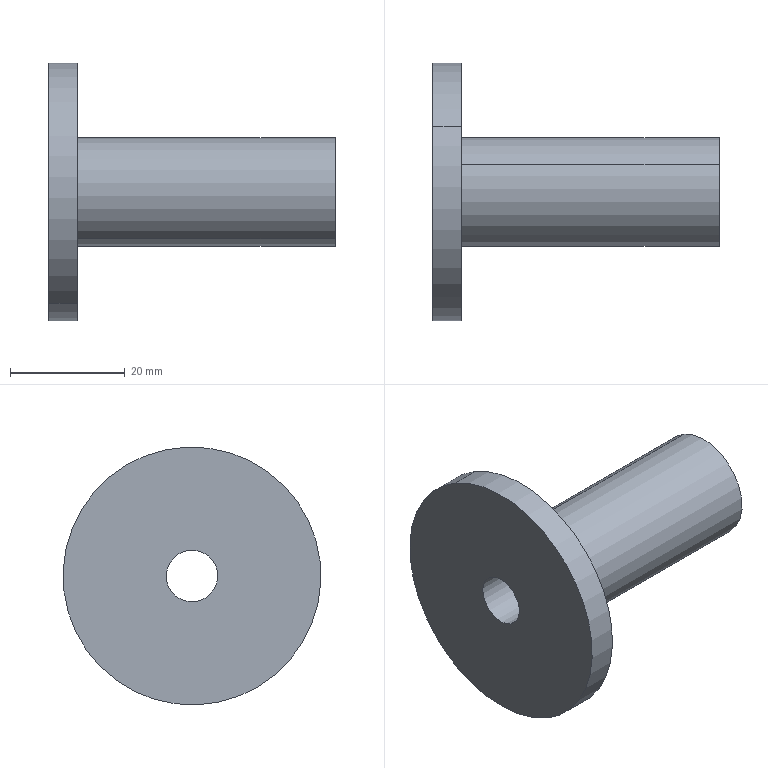Component | SolidWorks | ElectricalBoxAssembly2-1_MotorShaftSleeve2-1 | 1 solid | 9 faces | box 50 x 45 x 45 mm | volume 17530 mm3 | cylinder 6 | plane 3 | commonest cylinder face diameters 9 x2 19 x2 45 x2
build123d program:
from build123d import *

# Parameters (mm, degrees)
SKETCH1_R           = 22.5
BOSS_EXTRUDE1_DEPTH = 5
SKETCH2_R           = 9.5
BOSS_EXTRUDE2_DEPTH = 45
SKETCH3_R           = 4.5
CUT_EXTRUDE1_DEPTH  = 60.266


with BuildPart() as part:
    # Sketch1 → Boss-Extrude1 (new body)
    with BuildSketch(Plane.XY):
        Circle(SKETCH1_R)
    extrude(amount=BOSS_EXTRUDE1_DEPTH)

    # Sketch2 → Boss-Extrude2 (add)
    with BuildSketch(Plane.XY.offset(5)):
        with Locations(Location((0, 0, 0), (0, 0, 180))):
            Circle(SKETCH2_R)
    extrude(amount=BOSS_EXTRUDE2_DEPTH)

    # Sketch3 → Cut-Extrude1 (cut, through all)
    with BuildSketch(Plane(origin=(0, 0, 0), x_dir=(-1, 0, 0), z_dir=(0, 0, -1))):
        Circle(SKETCH3_R)
    extrude(amount=-CUT_EXTRUDE1_DEPTH, mode=Mode.SUBTRACT)


solid = part.part

# Placed as in the assembly
solid = solid.moved(Location((673.468, 214.666, 1526.399), (0, 90, 0)))
STEP:
#1=COLOUR_RGB('',0.7922,0.8196,0.9333);
#2=FILL_AREA_STYLE_COLOUR('',#1);
#3=FILL_AREA_STYLE('',(#2));
#4=SURFACE_STYLE_FILL_AREA(#3);
#5=SURFACE_SIDE_STYLE('',(#4));
#6=SURFACE_STYLE_USAGE(.BOTH.,#5);
#7=PRESENTATION_STYLE_ASSIGNMENT((#6));
#8=CARTESIAN_POINT('',(28.483,8.541,60.247));
#9=VERTEX_POINT('',#8);
#10=CARTESIAN_POINT('',(28.483,8.362,59.942));
#11=VERTEX_POINT('',#10);
#12=CARTESIAN_POINT('',(28.483,8.451,60.094));
#13=DIRECTION('',(-1.,0.,-0.));
#14=DIRECTION('',(0.,-0.5052,-0.863));
#15=AXIS2_PLACEMENT_3D('',#12,#13,#14);
#16=CIRCLE('',#15,0.1772);
#17=EDGE_CURVE('',#9,#11,#16,.T.);
#18=ORIENTED_EDGE('',*,*,#17,.F.);
#19=CARTESIAN_POINT('',(26.514,8.541,60.247));
#20=VERTEX_POINT('',#19);
#21=CARTESIAN_POINT('',(28.483,8.541,60.247));
#22=DIRECTION('',(-1.,0.,-0.));
#23=VECTOR('',#22,39.37);
#24=LINE('',#21,#23);
#25=EDGE_CURVE('',#9,#20,#24,.T.);
#26=ORIENTED_EDGE('',*,*,#25,.T.);
#27=CARTESIAN_POINT('',(26.514,8.362,59.942));
#28=VERTEX_POINT('',#27);
#29=CARTESIAN_POINT('',(26.514,8.451,60.094));
#30=DIRECTION('',(-1.,0.,-0.));
#31=DIRECTION('',(0.,-0.5052,-0.863));
#32=AXIS2_PLACEMENT_3D('',#29,#30,#31);
#33=CIRCLE('',#32,0.1772);
#34=EDGE_CURVE('',#20,#28,#33,.T.);
#35=ORIENTED_EDGE('',*,*,#34,.T.);
#36=CARTESIAN_POINT('',(28.483,8.362,59.942));
#37=DIRECTION('',(-1.,0.,-0.));
#38=VECTOR('',#37,39.37);
#39=LINE('',#36,#38);
#40=EDGE_CURVE('',#11,#28,#39,.T.);
#41=ORIENTED_EDGE('',*,*,#40,.F.);
#42=EDGE_LOOP('',(#18,#26,#35,#41));
#43=FACE_OUTER_BOUND('',#42,.T.);
#44=CARTESIAN_POINT('',(28.483,8.451,60.094));
#45=DIRECTION('',(-1.,0.,-0.));
#46=DIRECTION('',(0.,-0.5052,-0.863));
#47=AXIS2_PLACEMENT_3D('',#44,#45,#46);
#48=CYLINDRICAL_SURFACE('',#47,0.1772);
#49=ADVANCED_FACE('',(#43),#48,.F.);
#50=CARTESIAN_POINT('',(28.483,8.64,60.417));
#51=VERTEX_POINT('',#50);
#52=CARTESIAN_POINT('',(28.483,8.262,59.772));
#53=VERTEX_POINT('',#52);
#54=CARTESIAN_POINT('',(28.483,8.451,60.094));
#55=DIRECTION('',(1.,-0.,0.));
#56=DIRECTION('',(0.,0.5052,0.863));
#57=AXIS2_PLACEMENT_3D('',#54,#55,#56);
#58=CIRCLE('',#57,0.374);
#59=EDGE_CURVE('',#51,#53,#58,.T.);
#60=ORIENTED_EDGE('',*,*,#59,.F.);
#61=CARTESIAN_POINT('',(26.711,8.64,60.417));
#62=VERTEX_POINT('',#61);
#63=CARTESIAN_POINT('',(28.483,8.64,60.417));
#64=DIRECTION('',(-1.,0.,-0.));
#65=VECTOR('',#64,39.37);
#66=LINE('',#63,#65);
#67=EDGE_CURVE('',#51,#62,#66,.T.);
#68=ORIENTED_EDGE('',*,*,#67,.T.);
#69=CARTESIAN_POINT('',(26.711,8.262,59.772));
#70=VERTEX_POINT('',#69);
#71=CARTESIAN_POINT('',(26.711,8.451,60.094));
#72=DIRECTION('',(1.,-0.,0.));
#73=DIRECTION('',(0.,0.5052,0.863));
#74=AXIS2_PLACEMENT_3D('',#71,#72,#73);
#75=CIRCLE('',#74,0.374);
#76=EDGE_CURVE('',#62,#70,#75,.T.);
#77=ORIENTED_EDGE('',*,*,#76,.T.);
#78=CARTESIAN_POINT('',(28.483,8.262,59.772));
#79=DIRECTION('',(-1.,0.,-0.));
#80=VECTOR('',#79,39.37);
#81=LINE('',#78,#80);
#82=EDGE_CURVE('',#53,#70,#81,.T.);
#83=ORIENTED_EDGE('',*,*,#82,.F.);
#84=EDGE_LOOP('',(#60,#68,#77,#83));
#85=FACE_OUTER_BOUND('',#84,.T.);
#86=CARTESIAN_POINT('',(28.483,8.451,60.094));
#87=DIRECTION('',(-1.,0.,-0.));
#88=DIRECTION('',(0.,-0.5052,-0.863));
#89=AXIS2_PLACEMENT_3D('',#86,#87,#88);
#90=CYLINDRICAL_SURFACE('',#89,0.374);
#91=ADVANCED_FACE('',(#85),#90,.T.);
#92=CARTESIAN_POINT('',(26.711,8.899,60.859));
#93=VERTEX_POINT('',#92);
#94=CARTESIAN_POINT('',(26.711,8.004,59.33));
#95=VERTEX_POINT('',#94);
#96=CARTESIAN_POINT('',(26.711,8.451,60.094));
#97=DIRECTION('',(1.,-0.,0.));
#98=DIRECTION('',(0.,0.5052,0.863));
#99=AXIS2_PLACEMENT_3D('',#96,#97,#98);
#100=CIRCLE('',#99,0.8858);
#101=EDGE_CURVE('',#93,#95,#100,.T.);
#102=ORIENTED_EDGE('',*,*,#101,.F.);
#103=CARTESIAN_POINT('',(26.514,8.899,60.859));
#104=VERTEX_POINT('',#103);
#105=CARTESIAN_POINT('',(26.711,8.899,60.859));
#106=DIRECTION('',(-1.,0.,-0.));
#107=VECTOR('',#106,39.37);
#108=LINE('',#105,#107);
#109=EDGE_CURVE('',#93,#104,#108,.T.);
#110=ORIENTED_EDGE('',*,*,#109,.T.);
#111=CARTESIAN_POINT('',(26.514,8.004,59.33));
#112=VERTEX_POINT('',#111);
#113=CARTESIAN_POINT('',(26.514,8.451,60.094));
#114=DIRECTION('',(1.,-0.,0.));
#115=DIRECTION('',(0.,0.5052,0.863));
#116=AXIS2_PLACEMENT_3D('',#113,#114,#115);
#117=CIRCLE('',#116,0.8858);
#118=EDGE_CURVE('',#104,#112,#117,.T.);
#119=ORIENTED_EDGE('',*,*,#118,.T.);
#120=CARTESIAN_POINT('',(26.711,8.004,59.33));
#121=DIRECTION('',(-1.,0.,-0.));
#122=VECTOR('',#121,39.37);
#123=LINE('',#120,#122);
#124=EDGE_CURVE('',#95,#112,#123,.T.);
#125=ORIENTED_EDGE('',*,*,#124,.F.);
#126=EDGE_LOOP('',(#102,#110,#119,#125));
#127=FACE_OUTER_BOUND('',#126,.T.);
#128=CARTESIAN_POINT('',(26.711,8.451,60.094));
#129=DIRECTION('',(-1.,0.,-0.));
#130=DIRECTION('',(0.,-0.5052,-0.863));
#131=AXIS2_PLACEMENT_3D('',#128,#129,#130);
#132=CYLINDRICAL_SURFACE('',#131,0.8858);
#133=ADVANCED_FACE('',(#127),#132,.T.);
#134=ORIENTED_EDGE('',*,*,#109,.F.);
#135=CARTESIAN_POINT('',(26.711,8.451,60.094));
#136=DIRECTION('',(1.,-0.,0.));
#137=DIRECTION('',(0.,0.5052,0.863));
#138=AXIS2_PLACEMENT_3D('',#135,#136,#137);
#139=CIRCLE('',#138,0.8858);
#140=EDGE_CURVE('',#95,#93,#139,.T.);
#141=ORIENTED_EDGE('',*,*,#140,.F.);
#142=ORIENTED_EDGE('',*,*,#124,.T.);
#143=CARTESIAN_POINT('',(26.514,8.451,60.094));
#144=DIRECTION('',(1.,-0.,0.));
#145=DIRECTION('',(0.,0.5052,0.863));
#146=AXIS2_PLACEMENT_3D('',#143,#144,#145);
#147=CIRCLE('',#146,0.8858);
#148=EDGE_CURVE('',#112,#104,#147,.T.);
#149=ORIENTED_EDGE('',*,*,#148,.T.);
#150=EDGE_LOOP('',(#134,#141,#142,#149));
#151=FACE_OUTER_BOUND('',#150,.T.);
#152=CARTESIAN_POINT('',(26.711,8.451,60.094));
#153=DIRECTION('',(-1.,0.,-0.));
#154=DIRECTION('',(0.,-0.5052,-0.863));
#155=AXIS2_PLACEMENT_3D('',#152,#153,#154);
#156=CYLINDRICAL_SURFACE('',#155,0.8858);
#157=ADVANCED_FACE('',(#151),#156,.T.);
#158=CARTESIAN_POINT('',(26.711,8.451,60.094));
#159=DIRECTION('',(1.,-0.,0.));
#160=DIRECTION('',(0.,0.5052,0.863));
#161=AXIS2_PLACEMENT_3D('',#158,#159,#160);
#162=CIRCLE('',#161,0.374);
#163=EDGE_CURVE('',#70,#62,#162,.T.);
#164=ORIENTED_EDGE('',*,*,#163,.F.);
#165=ORIENTED_EDGE('',*,*,#76,.F.);
#166=EDGE_LOOP('',(#164,#165));
#167=FACE_BOUND('',#166,.T.);
#168=ORIENTED_EDGE('',*,*,#140,.T.);
#169=ORIENTED_EDGE('',*,*,#101,.T.);
#170=EDGE_LOOP('',(#168,#169));
#171=FACE_OUTER_BOUND('',#170,.T.);
#172=CARTESIAN_POINT('',(26.711,8.451,60.094));
#173=DIRECTION('',(1.,-0.,0.));
#174=DIRECTION('',(-0.,0.5052,0.863));
#175=AXIS2_PLACEMENT_3D('',#172,#173,#174);
#176=PLANE('',#175);
#177=ADVANCED_FACE('',(#167,#171),#176,.T.);
#178=CARTESIAN_POINT('',(26.514,8.451,60.094));
#179=DIRECTION('',(-1.,0.,-0.));
#180=DIRECTION('',(0.,-0.5052,-0.863));
#181=AXIS2_PLACEMENT_3D('',#178,#179,#180);
#182=CIRCLE('',#181,0.1772);
#183=EDGE_CURVE('',#28,#20,#182,.T.);
#184=ORIENTED_EDGE('',*,*,#183,.F.);
#185=ORIENTED_EDGE('',*,*,#34,.F.);
#186=EDGE_LOOP('',(#184,#185));
#187=FACE_BOUND('',#186,.T.);
#188=ORIENTED_EDGE('',*,*,#148,.F.);
#189=ORIENTED_EDGE('',*,*,#118,.F.);
#190=EDGE_LOOP('',(#188,#189));
#191=FACE_OUTER_BOUND('',#190,.T.);
#192=CARTESIAN_POINT('',(26.514,8.451,60.094));
#193=DIRECTION('',(1.,-0.,0.));
#194=DIRECTION('',(-0.,0.5052,0.863));
#195=AXIS2_PLACEMENT_3D('',#192,#193,#194);
#196=PLANE('',#195);
#197=ADVANCED_FACE('',(#187,#191),#196,.F.);
#198=ORIENTED_EDGE('',*,*,#67,.F.);
#199=CARTESIAN_POINT('',(28.483,8.451,60.094));
#200=DIRECTION('',(1.,-0.,0.));
#201=DIRECTION('',(0.,0.5052,0.863));
#202=AXIS2_PLACEMENT_3D('',#199,#200,#201);
#203=CIRCLE('',#202,0.374);
#204=EDGE_CURVE('',#53,#51,#203,.T.);
#205=ORIENTED_EDGE('',*,*,#204,.F.);
#206=ORIENTED_EDGE('',*,*,#82,.T.);
#207=ORIENTED_EDGE('',*,*,#163,.T.);
#208=EDGE_LOOP('',(#198,#205,#206,#207));
#209=FACE_OUTER_BOUND('',#208,.T.);
#210=CARTESIAN_POINT('',(28.483,8.451,60.094));
#211=DIRECTION('',(-1.,0.,-0.));
#212=DIRECTION('',(0.,-0.5052,-0.863));
#213=AXIS2_PLACEMENT_3D('',#210,#211,#212);
#214=CYLINDRICAL_SURFACE('',#213,0.374);
#215=ADVANCED_FACE('',(#209),#214,.T.);
#216=CARTESIAN_POINT('',(28.483,8.451,60.094));
#217=DIRECTION('',(-1.,0.,-0.));
#218=DIRECTION('',(0.,-0.5052,-0.863));
#219=AXIS2_PLACEMENT_3D('',#216,#217,#218);
#220=CIRCLE('',#219,0.1772);
#221=EDGE_CURVE('',#11,#9,#220,.T.);
#222=ORIENTED_EDGE('',*,*,#221,.T.);
#223=ORIENTED_EDGE('',*,*,#17,.T.);
#224=EDGE_LOOP('',(#222,#223));
#225=FACE_BOUND('',#224,.T.);
#226=ORIENTED_EDGE('',*,*,#204,.T.);
#227=ORIENTED_EDGE('',*,*,#59,.T.);
#228=EDGE_LOOP('',(#226,#227));
#229=FACE_OUTER_BOUND('',#228,.T.);
#230=CARTESIAN_POINT('',(28.483,8.451,60.094));
#231=DIRECTION('',(1.,-0.,0.));
#232=DIRECTION('',(-0.,0.5052,0.863));
#233=AXIS2_PLACEMENT_3D('',#230,#231,#232);
#234=PLANE('',#233);
#235=ADVANCED_FACE('',(#225,#229),#234,.T.);
#236=ORIENTED_EDGE('',*,*,#25,.F.);
#237=ORIENTED_EDGE('',*,*,#221,.F.);
#238=ORIENTED_EDGE('',*,*,#40,.T.);
#239=ORIENTED_EDGE('',*,*,#183,.T.);
#240=EDGE_LOOP('',(#236,#237,#238,#239));
#241=FACE_OUTER_BOUND('',#240,.T.);
#242=CARTESIAN_POINT('',(28.483,8.451,60.094));
#243=DIRECTION('',(-1.,0.,-0.));
#244=DIRECTION('',(0.,-0.5052,-0.863));
#245=AXIS2_PLACEMENT_3D('',#242,#243,#244);
#246=CYLINDRICAL_SURFACE('',#245,0.1772);
#247=ADVANCED_FACE('',(#241),#246,.F.);
#248=CLOSED_SHELL('',(#49,#91,#133,#157,#177,#197,#215,#235,#247));
#249=MANIFOLD_SOLID_BREP('',#248);
#250=STYLED_ITEM('',(#7),#249);
#251=(LENGTH_UNIT()NAMED_UNIT(*)SI_UNIT($,.METRE.));
#252=LENGTH_MEASURE_WITH_UNIT(LENGTH_MEASURE(0.0254),#251);
#253=DIMENSIONAL_EXPONENTS(1.,0.,0.,0.,0.,0.,0.);
#254=(CONVERSION_BASED_UNIT('',#252)LENGTH_UNIT()NAMED_UNIT(#253));
#255=UNCERTAINTY_MEASURE_WITH_UNIT(LENGTH_MEASURE(0.00001),#254,'','');
#256=(NAMED_UNIT(*)PLANE_ANGLE_UNIT()SI_UNIT($,.RADIAN.));
#257=(NAMED_UNIT(*)SI_UNIT($,.STERADIAN.)SOLID_ANGLE_UNIT());
#258=(GEOMETRIC_REPRESENTATION_CONTEXT(3)GLOBAL_UNCERTAINTY_ASSIGNED_CONTEXT((#255))GLOBAL_UNIT_ASSIGNED_CONTEXT((#254,#256,#257))REPRESENTATION_CONTEXT('',''));
#259=MECHANICAL_DESIGN_GEOMETRIC_PRESENTATION_REPRESENTATION('',(#250),#258);
#260=CARTESIAN_POINT('',(0.,0.,0.));
#261=DIRECTION('',(0.,0.,1.));
#262=DIRECTION('',(1.,0.,0.));
#263=AXIS2_PLACEMENT_3D('',#260,#261,#262);
#264=(LENGTH_UNIT()NAMED_UNIT(*)SI_UNIT($,.METRE.));
#265=LENGTH_MEASURE_WITH_UNIT(LENGTH_MEASURE(0.0254),#264);
#266=DIMENSIONAL_EXPONENTS(1.,0.,0.,0.,0.,0.,0.);
#267=(CONVERSION_BASED_UNIT('',#265)LENGTH_UNIT()NAMED_UNIT(#266));
#268=UNCERTAINTY_MEASURE_WITH_UNIT(LENGTH_MEASURE(0.00001),#267,'','');
#269=(NAMED_UNIT(*)PLANE_ANGLE_UNIT()SI_UNIT($,.RADIAN.));
#270=(NAMED_UNIT(*)SI_UNIT($,.STERADIAN.)SOLID_ANGLE_UNIT());
#271=(GEOMETRIC_REPRESENTATION_CONTEXT(3)GLOBAL_UNCERTAINTY_ASSIGNED_CONTEXT((#268))GLOBAL_UNIT_ASSIGNED_CONTEXT((#267,#269,#270))REPRESENTATION_CONTEXT('',''));
#272=ADVANCED_BREP_SHAPE_REPRESENTATION('',(#249,#263),#271);
#273=PRESENTATION_LAYER_ASSIGNMENT('','',(#250));